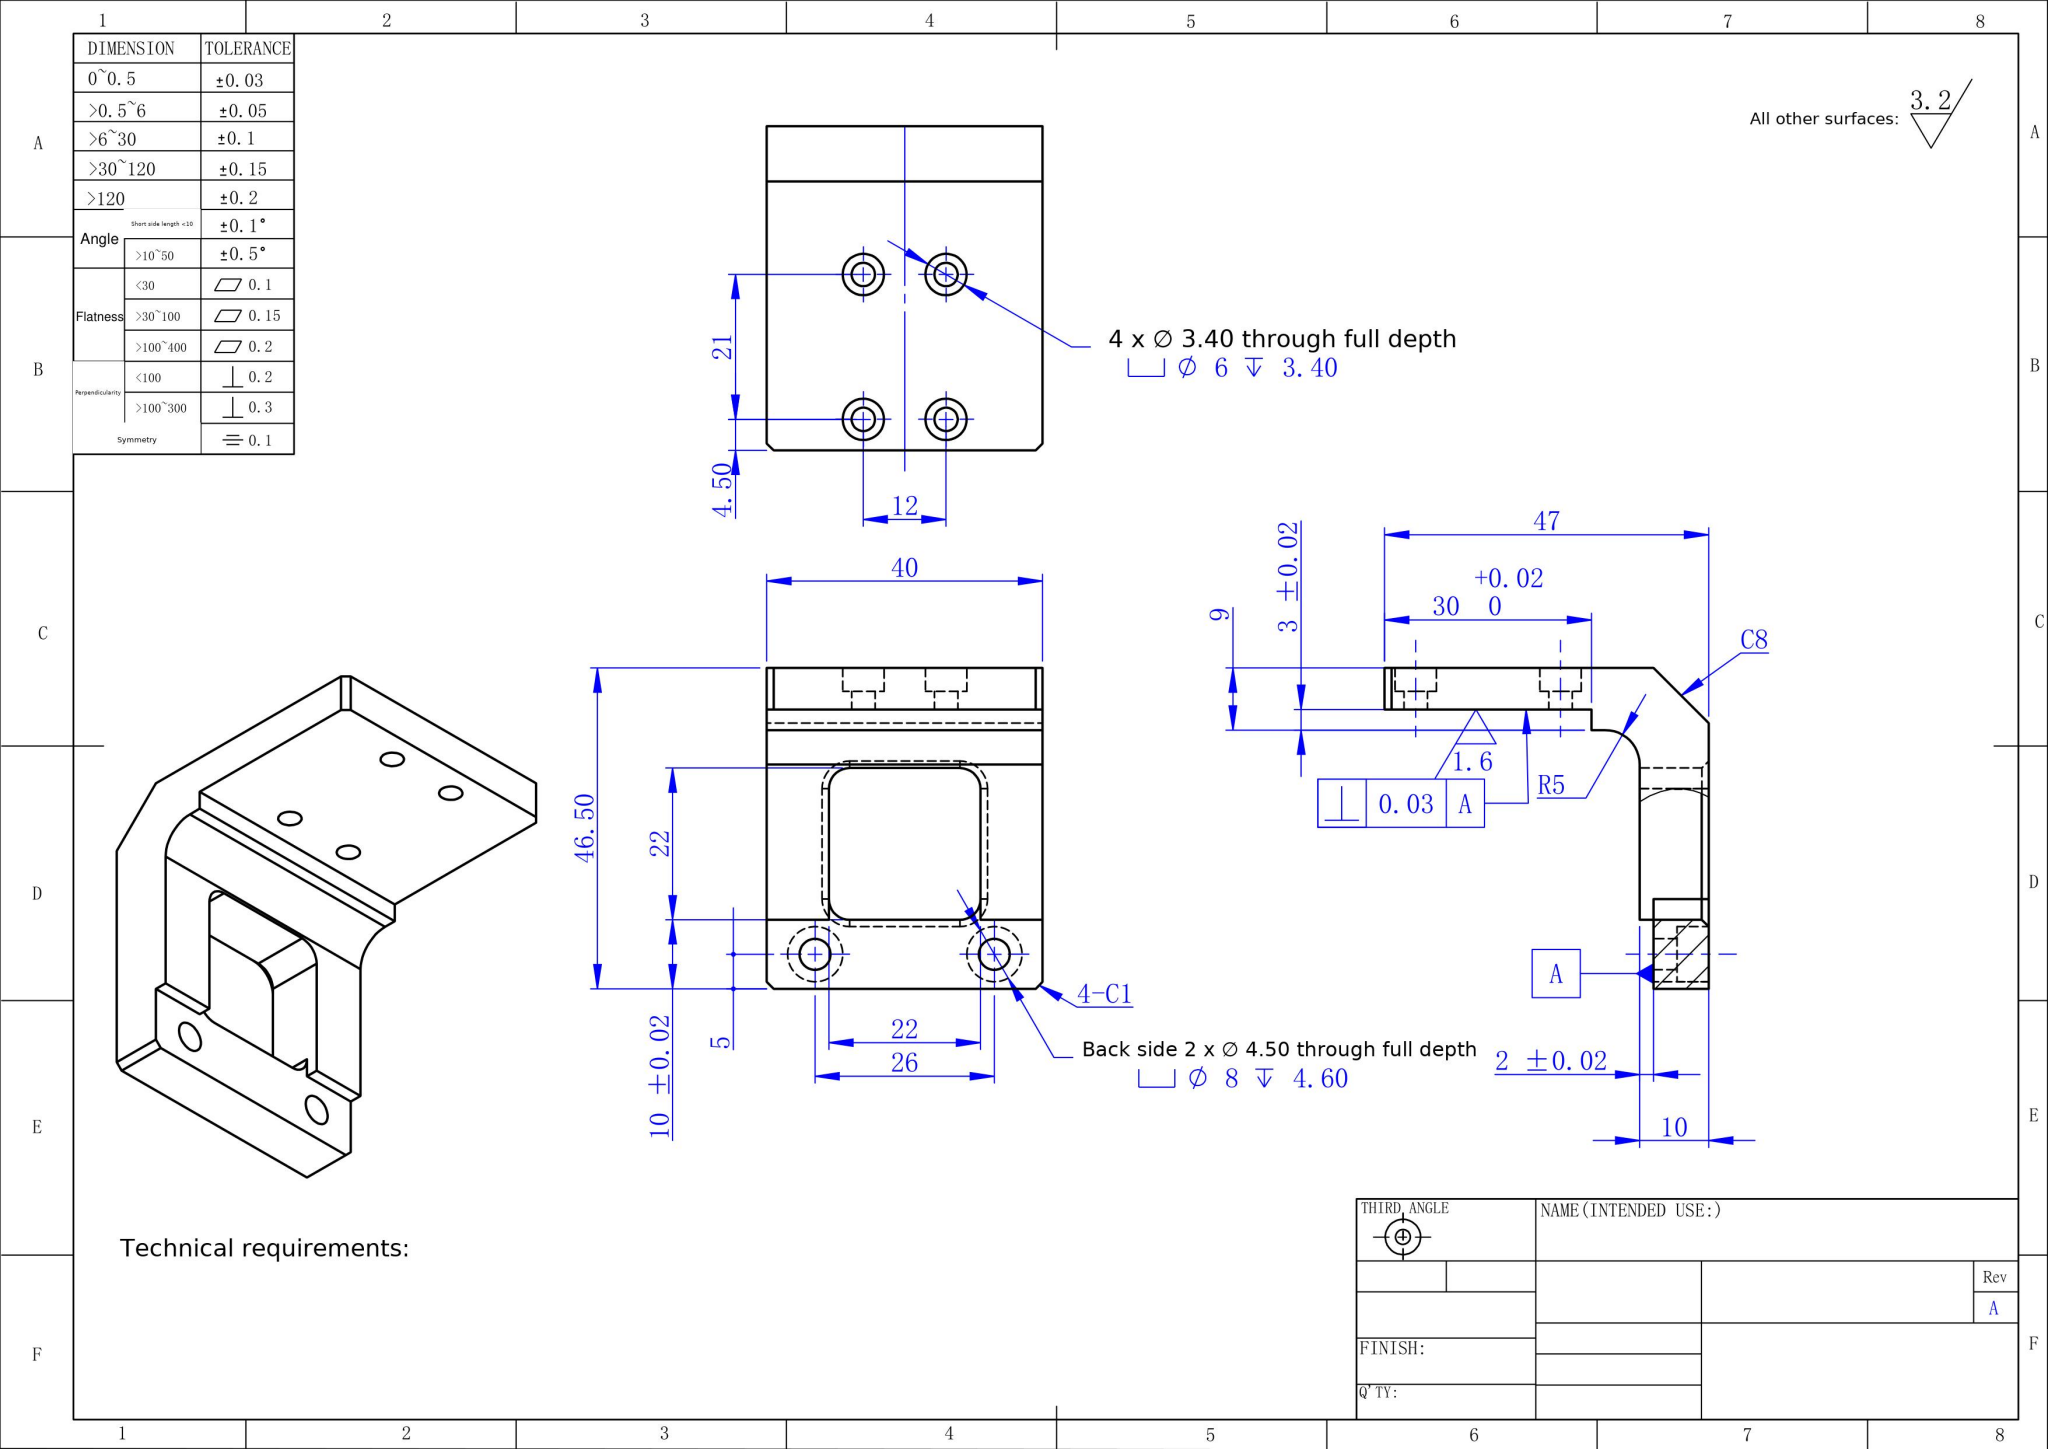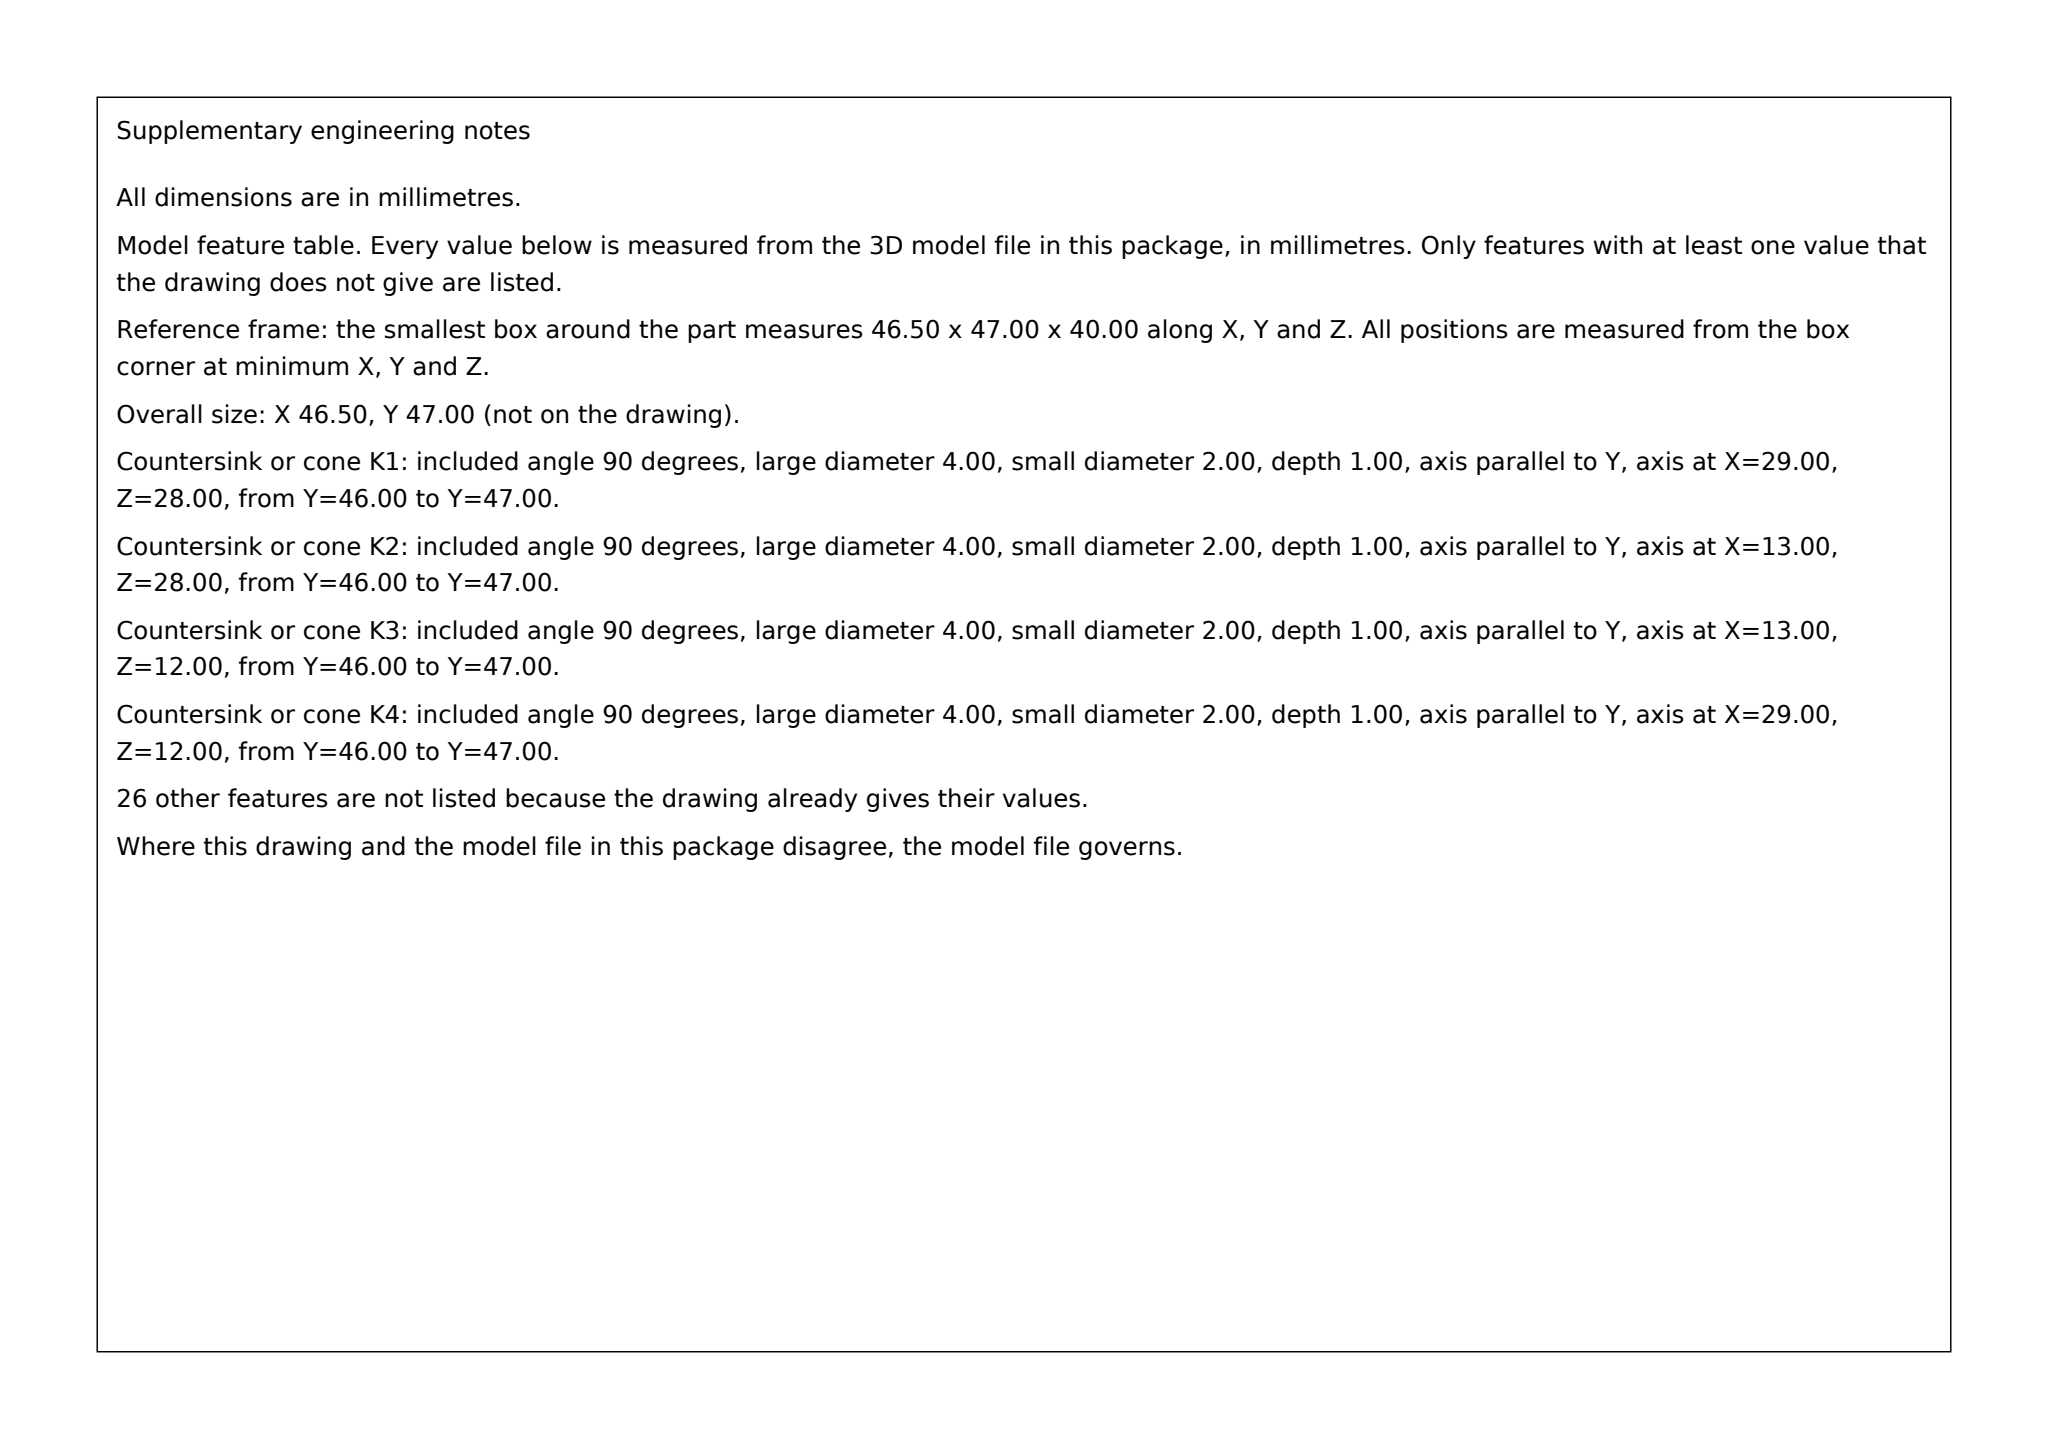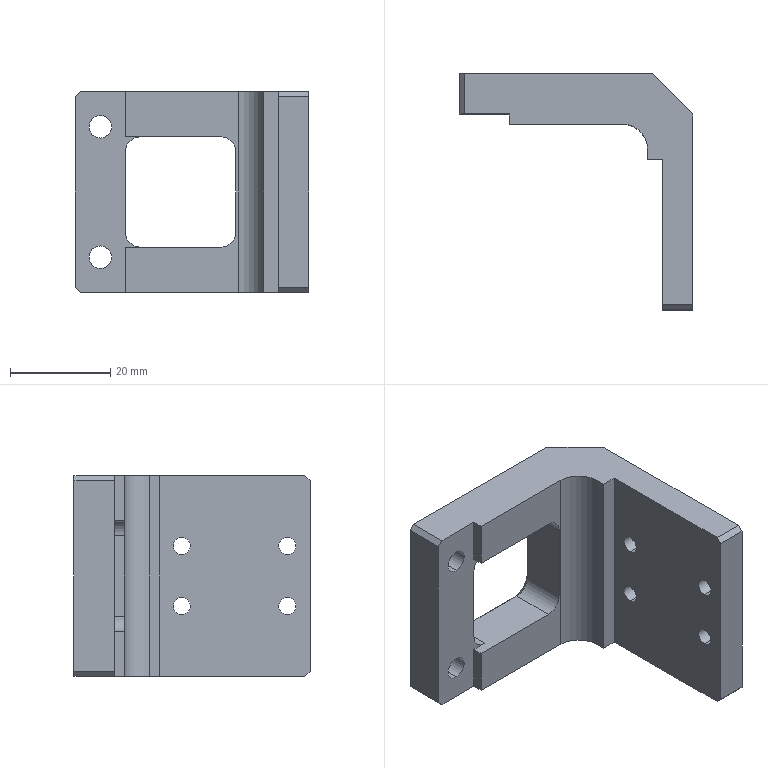Part | SolidWorks | mm | 1 solid | 65 faces | box 46.5 x 47 x 40 mm | volume 20578 mm3 | plane 32 | cylinder 29 | cone 4 | commonest cylinder face diameters 6 x12 3.4 x8 8 x4 4.5 x4 10 x1
build123d program:
from build123d import *

# Parameters (mm, degrees)
SKETCH2_W                                            = 40.5
SKETCH2_H                                            = 40
BOSS_EXTRUDE1_DEPTH                                  = 10
SKETCH4_W                                            = 40
SKETCH4_H                                            = 47
BOSS_EXTRUDE2_DEPTH                                  = 6
SKETCH5_W                                            = 10
SKETCH5_H                                            = 2
CUT_EXTRUDE2_DEPTH                                   = 61.482
HOLE_SIZE_ACCORDING_TO_THE_TYPE_OF_HEXAG_D           = 3.4
HOLE_SIZE_ACCORDING_TO_THE_TYPE_OF_HEXAG_CBORE_D     = 6
HOLE_SIZE_ACCORDING_TO_THE_TYPE_OF_HEXAG_CBORE_DEPTH = 3.4
HOLE_SIZE_ACCORDING_TO_THE_TYPE_OF_H_2_D             = 4.5
HOLE_SIZE_ACCORDING_TO_THE_TYPE_OF_H_2_CBORE_D       = 8
HOLE_SIZE_ACCORDING_TO_THE_TYPE_OF_H_2_CBORE_DEPTH   = 4.6
SKETCH10_W                                           = 3
SKETCH10_H                                           = 7
BOSS_EXTRUDE3_DEPTH                                  = 40
CHAMFER1_SIZE                                        = 1
CHAMFER2_SIZE                                        = 8
FILLET1_R                                            = 5
SKETCH3_W                                            = 22
SKETCH3_H                                            = 22
CUT_EXTRUDE3_DEPTH                                   = 58.429
FILLET2_R                                            = 3
CHAMFER3_SIZE                                        = 1


with BuildPart() as part:
    # Sketch2 → Boss-Extrude1 (new body)
    with BuildSketch(Plane(origin=(0, 0, 0), x_dir=(1, 0, 0), z_dir=(0, 1, 0))):
        Rectangle(SKETCH2_W, SKETCH2_H)
    extrude(amount=BOSS_EXTRUDE1_DEPTH)

    # Sketch4 → Boss-Extrude2 (add)
    with BuildSketch(Plane(origin=(20.25, 0, 0), x_dir=(0, 0, -1), z_dir=(1, 0, 0))):
        with Locations((0, -13.5)):
            Rectangle(SKETCH4_W, SKETCH4_H)
    extrude(amount=BOSS_EXTRUDE2_DEPTH)

    # Sketch5 → Cut-Extrude2 (cut, through all)
    with BuildSketch(Plane(origin=(0, 0, -20), x_dir=(-1, 0, 0), z_dir=(0, 0, -1))):
        with Locations((15.25, 1)):
            Rectangle(SKETCH5_W, SKETCH5_H)
    extrude(amount=-CUT_EXTRUDE2_DEPTH, mode=Mode.SUBTRACT)

    # Hole Size according to the type of Hexag (through all)
    with Locations(Plane(origin=(26.25, 0, 0), x_dir=(0, 0, -1), z_dir=(1, 0, 0))):
        with Locations((6, -11.5), (-6, -11.5), (6, -32.5), (-6, -32.5)):
            CounterBoreHole(HOLE_SIZE_ACCORDING_TO_THE_TYPE_OF_HEXAG_D / 2, HOLE_SIZE_ACCORDING_TO_THE_TYPE_OF_HEXAG_CBORE_D / 2, HOLE_SIZE_ACCORDING_TO_THE_TYPE_OF_HEXAG_CBORE_DEPTH)

    # Hole Size according to the type of H 2 (through all)
    with Locations(Plane(origin=(0, 10, 0), x_dir=(1, 0, 0), z_dir=(0, 1, 0))):
        with Locations((-15.25, 13), (-15.25, -13)):
            CounterBoreHole(HOLE_SIZE_ACCORDING_TO_THE_TYPE_OF_H_2_D / 2, HOLE_SIZE_ACCORDING_TO_THE_TYPE_OF_H_2_CBORE_D / 2, HOLE_SIZE_ACCORDING_TO_THE_TYPE_OF_H_2_CBORE_DEPTH)

    # Sketch10 → Boss-Extrude3 (add)
    with BuildSketch(Plane(origin=(0, 0, -20), x_dir=(-1, 0, 0), z_dir=(0, 0, -1))):
        with Locations((-18.75, -3.5)):
            Rectangle(SKETCH10_W, SKETCH10_H)
    extrude(amount=-BOSS_EXTRUDE3_DEPTH)

    # Chamfer1
    chamfer1_edges = [part.edges().sort_by_distance(p)[0] for p in [
        (23.25, -37, -20),
        (23.25, -37, 20),
        (-20.25, 6, -20),
        (-20.25, 6, 20),
    ]]
    chamfer(chamfer1_edges, length=CHAMFER1_SIZE)

    # Chamfer2
    chamfer2_edges = [part.edges().sort_by_distance(p)[0] for p in [
        (26.25, 10, 0),
    ]]
    chamfer(chamfer2_edges, length=CHAMFER2_SIZE)

    # Fillet1
    fillet1_edges = [part.edges().sort_by_distance(p)[0] for p in [
        (17.25, 0, 0),
    ]]
    fillet(fillet1_edges, radius=FILLET1_R)

    # Sketch3 → Cut-Extrude3 (cut, through all)
    with BuildSketch(Plane(origin=(0, 10, 0), x_dir=(1, 0, 0), z_dir=(0, 1, 0))):
        with Locations((0.75, 0)):
            Rectangle(SKETCH3_W, SKETCH3_H)
    extrude(amount=-CUT_EXTRUDE3_DEPTH, mode=Mode.SUBTRACT)

    # Fillet2
    fillet2_edges = [part.edges().sort_by_distance(p)[0] for p in [
        (11.75, 5, -11),
        (-10.25, 6, 11),
        (-10.25, 6, -11),
        (11.75, 5, 11),
    ]]
    fillet(fillet2_edges, radius=FILLET2_R)

    # Chamfer3
    chamfer3_edges = [part.edges().sort_by_distance(p)[0] for p in [
        (-10.25, 10, 0),
        (0.75, 10, -11),
        (0.75, 10, 11),
        (11.75, 10, 0),
        (-9.371, 10, -10.121),
        (-9.371, 10, 10.121),
        (10.871, 10, 10.121),
        (10.871, 10, -10.121),
    ]]
    chamfer(chamfer3_edges, length=CHAMFER3_SIZE)


solid = part.part